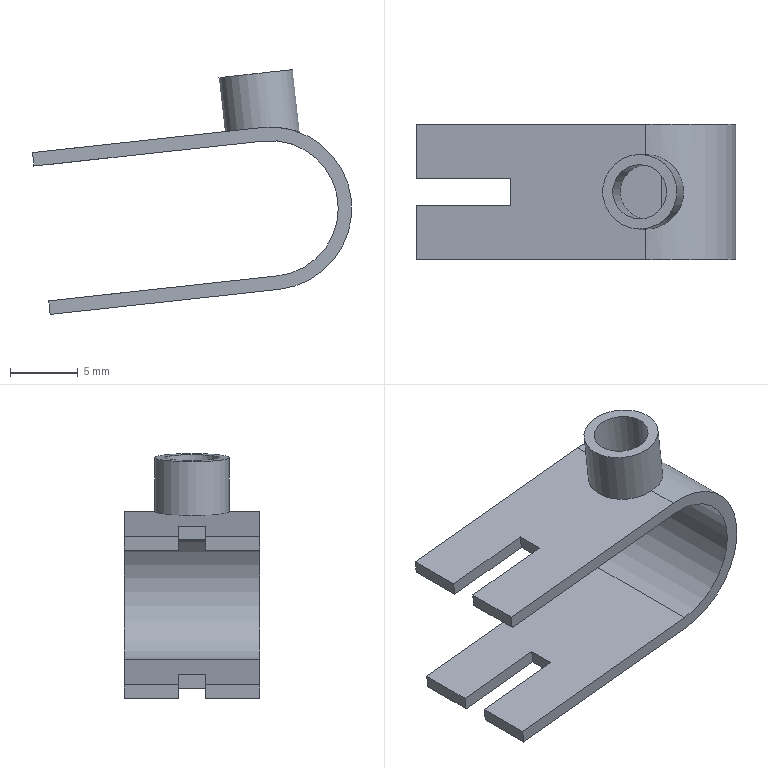Component | NX | LINK_3_LARGE_RING | 1 solid | 21 faces | volume 518 mm3 | plane 17 | cylinder 4 | commonest cylinder face diameters 12 x1 10 x1 5.5 x1 4 x1